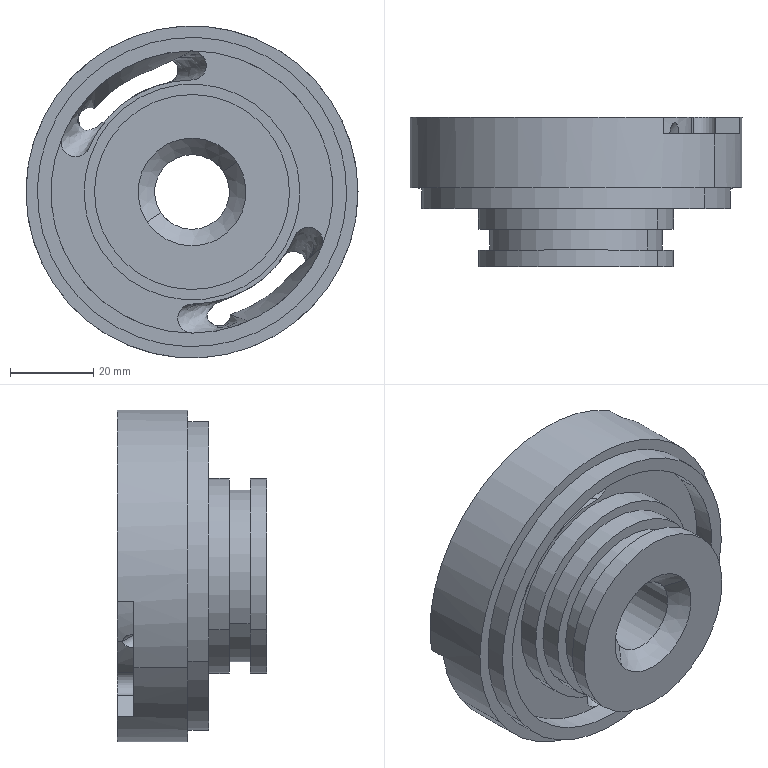Component | SolidWorks | 6-1 | 1 solid | 67 faces | volume 102114 mm3 | cylinder 43 | plane 16 | spline 6 | cone 2 | commonest cylinder face diameters 6 x12 4 x4 47 x4 57 x3 18 x2 29 x2 37 x2 74.52 x2